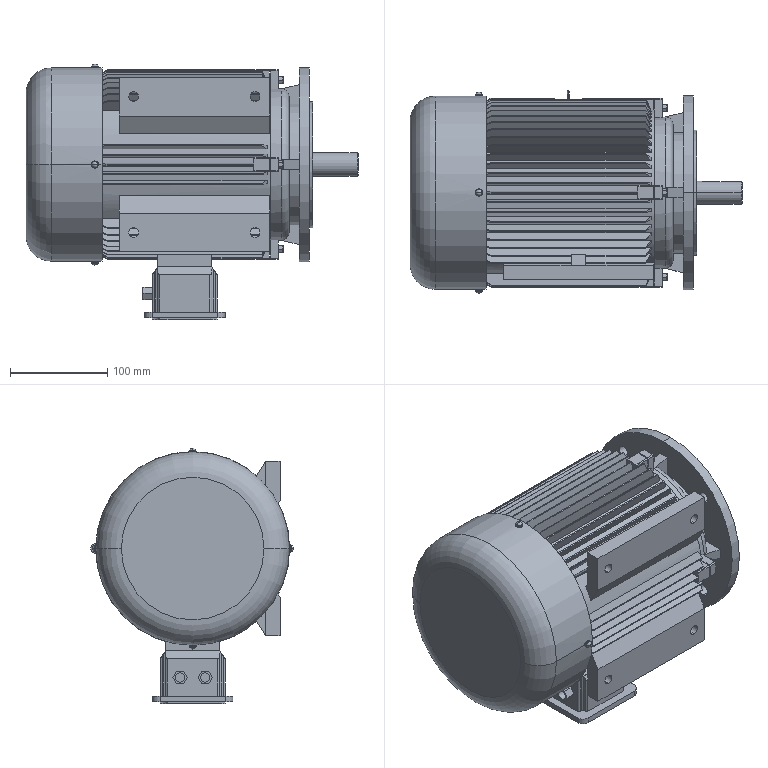Component | SolidWorks | FlangedMotorWithBase90L-1 | 1 solid | 679 faces | volume 6923625 mm3 | plane 421 | cone 138 | cylinder 98 | torus 14 | sphere 8 | commonest cylinder face diameters 171 x11 5.5 x9 12 x8 6.7 x8 7.5 x8 10 x8 15.75 x8 3.938 x6